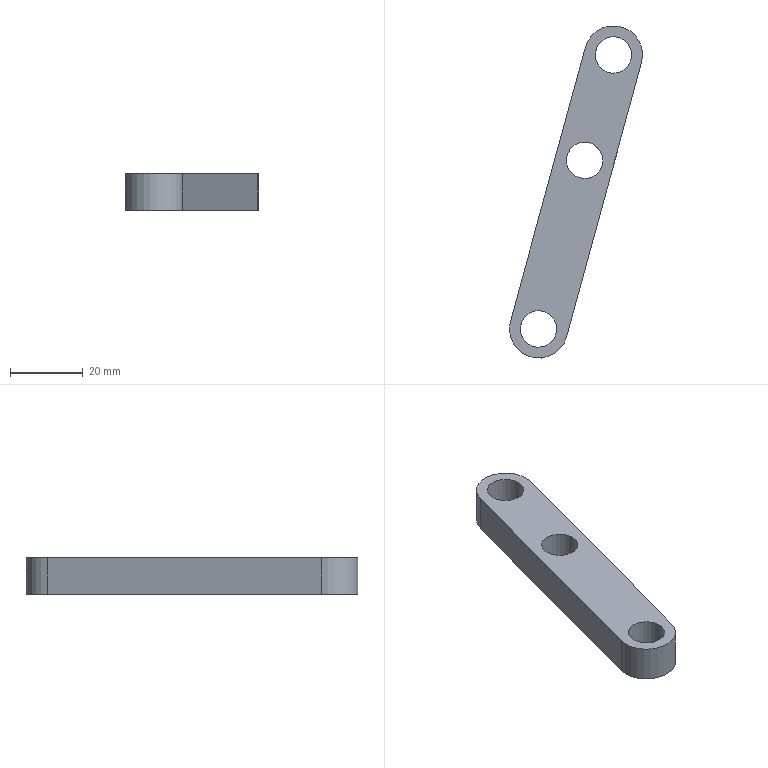Component | SolidWorks | ARocker-2 | 1 solid | 13 faces | box 36.56 x 91.24 x 10 mm | volume 12134 mm3 | cylinder 9 | plane 4 | commonest cylinder face diameters 10 x6 16 x3
build123d program:
from build123d import *

# Parameters (mm, degrees)
SKETCH1_R           = 5
BOSS_EXTRUDE1_DEPTH = 10


with BuildPart() as part:
    # Sketch1 → Boss-Extrude1 (new body)
    with BuildSketch(Plane.XY):
        with BuildLine():
            Line((-11.233, -5.015), (-60.126, 55.759))
            ThreePointArc((-60.126, 55.759), (-58.908, 67.007), (-47.66, 65.788))
            Line((-47.66, 65.788), (1.233, 5.015))
            ThreePointArc((1.233, 5.015), (0.01469, -6.233), (-11.233, -5.015))
        make_face()
        with Locations((-5, 0)):
            Circle(SKETCH1_R, mode=Mode.SUBTRACT)
        with Locations((-53.893, 60.774)):
            Circle(SKETCH1_R, mode=Mode.SUBTRACT)
        with Locations((-35.088, 37.399)):
            Circle(SKETCH1_R, mode=Mode.SUBTRACT)
    extrude(amount=BOSS_EXTRUDE1_DEPTH)


solid = part.part

# Placed as in the assembly
solid = solid.moved(Location((-69.375, -101.344, 137.182), (180, 0, 156.465)))
STEP:
#1=CARTESIAN_POINT('',(-2.168,-1.929,5.401));
#2=VERTEX_POINT('',#1);
#3=CARTESIAN_POINT('',(-1.937,-2.248,5.401));
#4=VERTEX_POINT('',#3);
#5=CARTESIAN_POINT('',(-2.053,-2.088,5.401));
#6=DIRECTION('',(-0.,0.,1.));
#7=DIRECTION('',(0.5864,-0.81,0.));
#8=AXIS2_PLACEMENT_3D('',#5,#6,#7);
#9=CIRCLE('',#8,0.1969);
#10=EDGE_CURVE('',#2,#4,#9,.T.);
#11=ORIENTED_EDGE('',*,*,#10,.T.);
#12=CARTESIAN_POINT('',(-1.937,-2.248,5.007));
#13=VERTEX_POINT('',#12);
#14=CARTESIAN_POINT('',(-1.937,-2.248,5.401));
#15=DIRECTION('',(0.,-0.,-1.));
#16=VECTOR('',#15,39.37);
#17=LINE('',#14,#16);
#18=EDGE_CURVE('',#4,#13,#17,.T.);
#19=ORIENTED_EDGE('',*,*,#18,.T.);
#20=CARTESIAN_POINT('',(-2.168,-1.929,5.007));
#21=VERTEX_POINT('',#20);
#22=CARTESIAN_POINT('',(-2.053,-2.088,5.007));
#23=DIRECTION('',(-0.,0.,1.));
#24=DIRECTION('',(0.5864,-0.81,0.));
#25=AXIS2_PLACEMENT_3D('',#22,#23,#24);
#26=CIRCLE('',#25,0.1969);
#27=EDGE_CURVE('',#21,#13,#26,.T.);
#28=ORIENTED_EDGE('',*,*,#27,.F.);
#29=CARTESIAN_POINT('',(-2.168,-1.929,5.401));
#30=DIRECTION('',(0.,-0.,-1.));
#31=VECTOR('',#30,39.37);
#32=LINE('',#29,#31);
#33=EDGE_CURVE('',#2,#21,#32,.T.);
#34=ORIENTED_EDGE('',*,*,#33,.F.);
#35=EDGE_LOOP('',(#11,#19,#28,#34));
#36=FACE_OUTER_BOUND('',#35,.T.);
#37=CARTESIAN_POINT('',(-2.053,-2.088,5.401));
#38=DIRECTION('',(0.,-0.,-1.));
#39=DIRECTION('',(-0.5864,0.81,0.));
#40=AXIS2_PLACEMENT_3D('',#37,#38,#39);
#41=CYLINDRICAL_SURFACE('',#40,0.1969);
#42=ADVANCED_FACE('',(#36),#41,.F.);
#43=CARTESIAN_POINT('',(-1.857,-0.7896,5.401));
#44=VERTEX_POINT('',#43);
#45=CARTESIAN_POINT('',(-1.626,-1.108,5.401));
#46=VERTEX_POINT('',#45);
#47=CARTESIAN_POINT('',(-1.741,-0.949,5.401));
#48=DIRECTION('',(-0.,0.,1.));
#49=DIRECTION('',(0.5864,-0.81,0.));
#50=AXIS2_PLACEMENT_3D('',#47,#48,#49);
#51=CIRCLE('',#50,0.1969);
#52=EDGE_CURVE('',#44,#46,#51,.T.);
#53=ORIENTED_EDGE('',*,*,#52,.T.);
#54=CARTESIAN_POINT('',(-1.626,-1.108,5.007));
#55=VERTEX_POINT('',#54);
#56=CARTESIAN_POINT('',(-1.626,-1.108,5.401));
#57=DIRECTION('',(0.,-0.,-1.));
#58=VECTOR('',#57,39.37);
#59=LINE('',#56,#58);
#60=EDGE_CURVE('',#46,#55,#59,.T.);
#61=ORIENTED_EDGE('',*,*,#60,.T.);
#62=CARTESIAN_POINT('',(-1.857,-0.7896,5.007));
#63=VERTEX_POINT('',#62);
#64=CARTESIAN_POINT('',(-1.741,-0.949,5.007));
#65=DIRECTION('',(-0.,0.,1.));
#66=DIRECTION('',(0.5864,-0.81,0.));
#67=AXIS2_PLACEMENT_3D('',#64,#65,#66);
#68=CIRCLE('',#67,0.1969);
#69=EDGE_CURVE('',#63,#55,#68,.T.);
#70=ORIENTED_EDGE('',*,*,#69,.F.);
#71=CARTESIAN_POINT('',(-1.857,-0.7896,5.401));
#72=DIRECTION('',(0.,-0.,-1.));
#73=VECTOR('',#72,39.37);
#74=LINE('',#71,#73);
#75=EDGE_CURVE('',#44,#63,#74,.T.);
#76=ORIENTED_EDGE('',*,*,#75,.F.);
#77=EDGE_LOOP('',(#53,#61,#70,#76));
#78=FACE_OUTER_BOUND('',#77,.T.);
#79=CARTESIAN_POINT('',(-1.741,-0.949,5.401));
#80=DIRECTION('',(0.,-0.,-1.));
#81=DIRECTION('',(-0.5864,0.81,0.));
#82=AXIS2_PLACEMENT_3D('',#79,#80,#81);
#83=CYLINDRICAL_SURFACE('',#82,0.1969);
#84=ADVANCED_FACE('',(#78),#83,.F.);
#85=CARTESIAN_POINT('',(-2.666,-3.752,5.401));
#86=VERTEX_POINT('',#85);
#87=CARTESIAN_POINT('',(-2.435,-4.071,5.401));
#88=VERTEX_POINT('',#87);
#89=CARTESIAN_POINT('',(-2.551,-3.911,5.401));
#90=DIRECTION('',(-0.,0.,1.));
#91=DIRECTION('',(0.5864,-0.81,0.));
#92=AXIS2_PLACEMENT_3D('',#89,#90,#91);
#93=CIRCLE('',#92,0.1969);
#94=EDGE_CURVE('',#86,#88,#93,.T.);
#95=ORIENTED_EDGE('',*,*,#94,.T.);
#96=CARTESIAN_POINT('',(-2.435,-4.071,5.007));
#97=VERTEX_POINT('',#96);
#98=CARTESIAN_POINT('',(-2.435,-4.071,5.401));
#99=DIRECTION('',(0.,-0.,-1.));
#100=VECTOR('',#99,39.37);
#101=LINE('',#98,#100);
#102=EDGE_CURVE('',#88,#97,#101,.T.);
#103=ORIENTED_EDGE('',*,*,#102,.T.);
#104=CARTESIAN_POINT('',(-2.666,-3.752,5.007));
#105=VERTEX_POINT('',#104);
#106=CARTESIAN_POINT('',(-2.551,-3.911,5.007));
#107=DIRECTION('',(-0.,0.,1.));
#108=DIRECTION('',(0.5864,-0.81,0.));
#109=AXIS2_PLACEMENT_3D('',#106,#107,#108);
#110=CIRCLE('',#109,0.1969);
#111=EDGE_CURVE('',#105,#97,#110,.T.);
#112=ORIENTED_EDGE('',*,*,#111,.F.);
#113=CARTESIAN_POINT('',(-2.666,-3.752,5.401));
#114=DIRECTION('',(0.,-0.,-1.));
#115=VECTOR('',#114,39.37);
#116=LINE('',#113,#115);
#117=EDGE_CURVE('',#86,#105,#116,.T.);
#118=ORIENTED_EDGE('',*,*,#117,.F.);
#119=EDGE_LOOP('',(#95,#103,#112,#118));
#120=FACE_OUTER_BOUND('',#119,.T.);
#121=CARTESIAN_POINT('',(-2.551,-3.911,5.401));
#122=DIRECTION('',(0.,-0.,-1.));
#123=DIRECTION('',(-0.5864,0.81,0.));
#124=AXIS2_PLACEMENT_3D('',#121,#122,#123);
#125=CYLINDRICAL_SURFACE('',#124,0.1969);
#126=ADVANCED_FACE('',(#120),#125,.F.);
#127=CARTESIAN_POINT('',(-1.926,-0.6939,5.401));
#128=VERTEX_POINT('',#127);
#129=CARTESIAN_POINT('',(-2.045,-0.866,5.401));
#130=VERTEX_POINT('',#129);
#131=CARTESIAN_POINT('',(-1.741,-0.949,5.401));
#132=DIRECTION('',(-0.,0.,1.));
#133=DIRECTION('',(0.5864,-0.81,0.));
#134=AXIS2_PLACEMENT_3D('',#131,#132,#133);
#135=CIRCLE('',#134,0.315);
#136=EDGE_CURVE('',#128,#130,#135,.T.);
#137=ORIENTED_EDGE('',*,*,#136,.F.);
#138=CARTESIAN_POINT('',(-1.926,-0.6939,5.007));
#139=VERTEX_POINT('',#138);
#140=CARTESIAN_POINT('',(-1.926,-0.6939,5.401));
#141=DIRECTION('',(0.,-0.,-1.));
#142=VECTOR('',#141,39.37);
#143=LINE('',#140,#142);
#144=EDGE_CURVE('',#128,#139,#143,.T.);
#145=ORIENTED_EDGE('',*,*,#144,.T.);
#146=CARTESIAN_POINT('',(-2.045,-0.866,5.007));
#147=VERTEX_POINT('',#146);
#148=CARTESIAN_POINT('',(-1.741,-0.949,5.007));
#149=DIRECTION('',(-0.,0.,1.));
#150=DIRECTION('',(0.5864,-0.81,0.));
#151=AXIS2_PLACEMENT_3D('',#148,#149,#150);
#152=CIRCLE('',#151,0.315);
#153=EDGE_CURVE('',#139,#147,#152,.T.);
#154=ORIENTED_EDGE('',*,*,#153,.T.);
#155=CARTESIAN_POINT('',(-2.045,-0.866,5.401));
#156=DIRECTION('',(0.,-0.,-1.));
#157=VECTOR('',#156,39.37);
#158=LINE('',#155,#157);
#159=EDGE_CURVE('',#130,#147,#158,.T.);
#160=ORIENTED_EDGE('',*,*,#159,.F.);
#161=EDGE_LOOP('',(#137,#145,#154,#160));
#162=FACE_OUTER_BOUND('',#161,.T.);
#163=CARTESIAN_POINT('',(-1.741,-0.949,5.401));
#164=DIRECTION('',(0.,-0.,-1.));
#165=DIRECTION('',(-0.5864,0.81,0.));
#166=AXIS2_PLACEMENT_3D('',#163,#164,#165);
#167=CYLINDRICAL_SURFACE('',#166,0.315);
#168=ADVANCED_FACE('',(#162),#167,.T.);
#169=ORIENTED_EDGE('',*,*,#52,.F.);
#170=CARTESIAN_POINT('',(-1.741,-0.949,5.401));
#171=DIRECTION('',(-0.,0.,1.));
#172=DIRECTION('',(0.5864,-0.81,0.));
#173=AXIS2_PLACEMENT_3D('',#170,#171,#172);
#174=CIRCLE('',#173,0.1969);
#175=EDGE_CURVE('',#46,#44,#174,.T.);
#176=ORIENTED_EDGE('',*,*,#175,.F.);
#177=EDGE_LOOP('',(#169,#176));
#178=FACE_BOUND('',#177,.T.);
#179=CARTESIAN_POINT('',(-2.855,-3.828,5.401));
#180=VERTEX_POINT('',#179);
#181=CARTESIAN_POINT('',(-2.247,-3.994,5.401));
#182=VERTEX_POINT('',#181);
#183=CARTESIAN_POINT('',(-2.551,-3.911,5.401));
#184=DIRECTION('',(-0.,0.,1.));
#185=DIRECTION('',(0.5864,-0.81,0.));
#186=AXIS2_PLACEMENT_3D('',#183,#184,#185);
#187=CIRCLE('',#186,0.315);
#188=EDGE_CURVE('',#180,#182,#187,.T.);
#189=ORIENTED_EDGE('',*,*,#188,.T.);
#190=CARTESIAN_POINT('',(-1.438,-1.032,5.401));
#191=VERTEX_POINT('',#190);
#192=CARTESIAN_POINT('',(-2.247,-3.994,5.401));
#193=DIRECTION('',(0.2636,0.9646,-0.));
#194=VECTOR('',#193,39.37);
#195=LINE('',#192,#194);
#196=EDGE_CURVE('',#182,#191,#195,.T.);
#197=ORIENTED_EDGE('',*,*,#196,.T.);
#198=CARTESIAN_POINT('',(-1.741,-0.949,5.401));
#199=DIRECTION('',(-0.,0.,1.));
#200=DIRECTION('',(0.5864,-0.81,0.));
#201=AXIS2_PLACEMENT_3D('',#198,#199,#200);
#202=CIRCLE('',#201,0.315);
#203=EDGE_CURVE('',#191,#128,#202,.T.);
#204=ORIENTED_EDGE('',*,*,#203,.T.);
#205=ORIENTED_EDGE('',*,*,#136,.T.);
#206=CARTESIAN_POINT('',(-2.855,-3.828,5.401));
#207=DIRECTION('',(-0.2636,-0.9646,0.));
#208=VECTOR('',#207,39.37);
#209=LINE('',#206,#208);
#210=EDGE_CURVE('',#130,#180,#209,.T.);
#211=ORIENTED_EDGE('',*,*,#210,.T.);
#212=EDGE_LOOP('',(#189,#197,#204,#205,#211));
#213=FACE_OUTER_BOUND('',#212,.T.);
#214=ORIENTED_EDGE('',*,*,#94,.F.);
#215=CARTESIAN_POINT('',(-2.551,-3.911,5.401));
#216=DIRECTION('',(-0.,0.,1.));
#217=DIRECTION('',(0.5864,-0.81,0.));
#218=AXIS2_PLACEMENT_3D('',#215,#216,#217);
#219=CIRCLE('',#218,0.1969);
#220=EDGE_CURVE('',#88,#86,#219,.T.);
#221=ORIENTED_EDGE('',*,*,#220,.F.);
#222=EDGE_LOOP('',(#214,#221));
#223=FACE_BOUND('',#222,.T.);
#224=ORIENTED_EDGE('',*,*,#10,.F.);
#225=CARTESIAN_POINT('',(-2.053,-2.088,5.401));
#226=DIRECTION('',(-0.,0.,1.));
#227=DIRECTION('',(0.5864,-0.81,0.));
#228=AXIS2_PLACEMENT_3D('',#225,#226,#227);
#229=CIRCLE('',#228,0.1969);
#230=EDGE_CURVE('',#4,#2,#229,.T.);
#231=ORIENTED_EDGE('',*,*,#230,.F.);
#232=EDGE_LOOP('',(#224,#231));
#233=FACE_BOUND('',#232,.T.);
#234=CARTESIAN_POINT('',(-2.551,-3.911,5.401));
#235=DIRECTION('',(-0.,0.,1.));
#236=DIRECTION('',(0.5864,-0.81,0.));
#237=AXIS2_PLACEMENT_3D('',#234,#235,#236);
#238=PLANE('',#237);
#239=ADVANCED_FACE('',(#178,#213,#223,#233),#238,.T.);
#240=CARTESIAN_POINT('',(-2.855,-3.828,5.007));
#241=VERTEX_POINT('',#240);
#242=CARTESIAN_POINT('',(-2.247,-3.994,5.007));
#243=VERTEX_POINT('',#242);
#244=CARTESIAN_POINT('',(-2.551,-3.911,5.007));
#245=DIRECTION('',(-0.,0.,1.));
#246=DIRECTION('',(0.5864,-0.81,0.));
#247=AXIS2_PLACEMENT_3D('',#244,#245,#246);
#248=CIRCLE('',#247,0.315);
#249=EDGE_CURVE('',#241,#243,#248,.T.);
#250=ORIENTED_EDGE('',*,*,#249,.F.);
#251=CARTESIAN_POINT('',(-2.855,-3.828,5.007));
#252=DIRECTION('',(-0.2636,-0.9646,0.));
#253=VECTOR('',#252,39.37);
#254=LINE('',#251,#253);
#255=EDGE_CURVE('',#147,#241,#254,.T.);
#256=ORIENTED_EDGE('',*,*,#255,.F.);
#257=ORIENTED_EDGE('',*,*,#153,.F.);
#258=CARTESIAN_POINT('',(-1.438,-1.032,5.007));
#259=VERTEX_POINT('',#258);
#260=CARTESIAN_POINT('',(-1.741,-0.949,5.007));
#261=DIRECTION('',(-0.,0.,1.));
#262=DIRECTION('',(0.5864,-0.81,0.));
#263=AXIS2_PLACEMENT_3D('',#260,#261,#262);
#264=CIRCLE('',#263,0.315);
#265=EDGE_CURVE('',#259,#139,#264,.T.);
#266=ORIENTED_EDGE('',*,*,#265,.F.);
#267=CARTESIAN_POINT('',(-2.247,-3.994,5.007));
#268=DIRECTION('',(0.2636,0.9646,-0.));
#269=VECTOR('',#268,39.37);
#270=LINE('',#267,#269);
#271=EDGE_CURVE('',#243,#259,#270,.T.);
#272=ORIENTED_EDGE('',*,*,#271,.F.);
#273=EDGE_LOOP('',(#250,#256,#257,#266,#272));
#274=FACE_OUTER_BOUND('',#273,.T.);
#275=ORIENTED_EDGE('',*,*,#111,.T.);
#276=CARTESIAN_POINT('',(-2.551,-3.911,5.007));
#277=DIRECTION('',(-0.,0.,1.));
#278=DIRECTION('',(0.5864,-0.81,0.));
#279=AXIS2_PLACEMENT_3D('',#276,#277,#278);
#280=CIRCLE('',#279,0.1969);
#281=EDGE_CURVE('',#97,#105,#280,.T.);
#282=ORIENTED_EDGE('',*,*,#281,.T.);
#283=EDGE_LOOP('',(#275,#282));
#284=FACE_BOUND('',#283,.T.);
#285=ORIENTED_EDGE('',*,*,#69,.T.);
#286=CARTESIAN_POINT('',(-1.741,-0.949,5.007));
#287=DIRECTION('',(-0.,0.,1.));
#288=DIRECTION('',(0.5864,-0.81,0.));
#289=AXIS2_PLACEMENT_3D('',#286,#287,#288);
#290=CIRCLE('',#289,0.1969);
#291=EDGE_CURVE('',#55,#63,#290,.T.);
#292=ORIENTED_EDGE('',*,*,#291,.T.);
#293=EDGE_LOOP('',(#285,#292));
#294=FACE_BOUND('',#293,.T.);
#295=ORIENTED_EDGE('',*,*,#27,.T.);
#296=CARTESIAN_POINT('',(-2.053,-2.088,5.007));
#297=DIRECTION('',(-0.,0.,1.));
#298=DIRECTION('',(0.5864,-0.81,0.));
#299=AXIS2_PLACEMENT_3D('',#296,#297,#298);
#300=CIRCLE('',#299,0.1969);
#301=EDGE_CURVE('',#13,#21,#300,.T.);
#302=ORIENTED_EDGE('',*,*,#301,.T.);
#303=EDGE_LOOP('',(#295,#302));
#304=FACE_BOUND('',#303,.T.);
#305=CARTESIAN_POINT('',(-2.551,-3.911,5.007));
#306=DIRECTION('',(-0.,0.,1.));
#307=DIRECTION('',(0.5864,-0.81,0.));
#308=AXIS2_PLACEMENT_3D('',#305,#306,#307);
#309=PLANE('',#308);
#310=ADVANCED_FACE('',(#274,#284,#294,#304),#309,.F.);
#311=ORIENTED_EDGE('',*,*,#249,.T.);
#312=CARTESIAN_POINT('',(-2.247,-3.994,5.401));
#313=DIRECTION('',(0.,-0.,-1.));
#314=VECTOR('',#313,39.37);
#315=LINE('',#312,#314);
#316=EDGE_CURVE('',#182,#243,#315,.T.);
#317=ORIENTED_EDGE('',*,*,#316,.F.);
#318=ORIENTED_EDGE('',*,*,#188,.F.);
#319=CARTESIAN_POINT('',(-2.855,-3.828,5.401));
#320=DIRECTION('',(0.,-0.,-1.));
#321=VECTOR('',#320,39.37);
#322=LINE('',#319,#321);
#323=EDGE_CURVE('',#180,#241,#322,.T.);
#324=ORIENTED_EDGE('',*,*,#323,.T.);
#325=EDGE_LOOP('',(#311,#317,#318,#324));
#326=FACE_OUTER_BOUND('',#325,.T.);
#327=CARTESIAN_POINT('',(-2.551,-3.911,5.401));
#328=DIRECTION('',(0.,-0.,-1.));
#329=DIRECTION('',(-0.5864,0.81,0.));
#330=AXIS2_PLACEMENT_3D('',#327,#328,#329);
#331=CYLINDRICAL_SURFACE('',#330,0.315);
#332=ADVANCED_FACE('',(#326),#331,.T.);
#333=ORIENTED_EDGE('',*,*,#271,.T.);
#334=CARTESIAN_POINT('',(-1.438,-1.032,5.401));
#335=DIRECTION('',(0.,-0.,-1.));
#336=VECTOR('',#335,39.37);
#337=LINE('',#334,#336);
#338=EDGE_CURVE('',#191,#259,#337,.T.);
#339=ORIENTED_EDGE('',*,*,#338,.F.);
#340=ORIENTED_EDGE('',*,*,#196,.F.);
#341=ORIENTED_EDGE('',*,*,#316,.T.);
#342=EDGE_LOOP('',(#333,#339,#340,#341));
#343=FACE_OUTER_BOUND('',#342,.T.);
#344=CARTESIAN_POINT('',(-2.247,-3.994,5.401));
#345=DIRECTION('',(-0.9646,0.2636,-0.));
#346=DIRECTION('',(-0.2636,-0.9646,0.));
#347=AXIS2_PLACEMENT_3D('',#344,#345,#346);
#348=PLANE('',#347);
#349=ADVANCED_FACE('',(#343),#348,.F.);
#350=ORIENTED_EDGE('',*,*,#144,.F.);
#351=ORIENTED_EDGE('',*,*,#203,.F.);
#352=ORIENTED_EDGE('',*,*,#338,.T.);
#353=ORIENTED_EDGE('',*,*,#265,.T.);
#354=EDGE_LOOP('',(#350,#351,#352,#353));
#355=FACE_OUTER_BOUND('',#354,.T.);
#356=CARTESIAN_POINT('',(-1.741,-0.949,5.401));
#357=DIRECTION('',(0.,-0.,-1.));
#358=DIRECTION('',(-0.5864,0.81,0.));
#359=AXIS2_PLACEMENT_3D('',#356,#357,#358);
#360=CYLINDRICAL_SURFACE('',#359,0.315);
#361=ADVANCED_FACE('',(#355),#360,.T.);
#362=ORIENTED_EDGE('',*,*,#255,.T.);
#363=ORIENTED_EDGE('',*,*,#323,.F.);
#364=ORIENTED_EDGE('',*,*,#210,.F.);
#365=ORIENTED_EDGE('',*,*,#159,.T.);
#366=EDGE_LOOP('',(#362,#363,#364,#365));
#367=FACE_OUTER_BOUND('',#366,.T.);
#368=CARTESIAN_POINT('',(-2.855,-3.828,5.401));
#369=DIRECTION('',(0.9646,-0.2636,0.));
#370=DIRECTION('',(0.2636,0.9646,-0.));
#371=AXIS2_PLACEMENT_3D('',#368,#369,#370);
#372=PLANE('',#371);
#373=ADVANCED_FACE('',(#367),#372,.F.);
#374=ORIENTED_EDGE('',*,*,#102,.F.);
#375=ORIENTED_EDGE('',*,*,#220,.T.);
#376=ORIENTED_EDGE('',*,*,#117,.T.);
#377=ORIENTED_EDGE('',*,*,#281,.F.);
#378=EDGE_LOOP('',(#374,#375,#376,#377));
#379=FACE_OUTER_BOUND('',#378,.T.);
#380=CARTESIAN_POINT('',(-2.551,-3.911,5.401));
#381=DIRECTION('',(0.,-0.,-1.));
#382=DIRECTION('',(-0.5864,0.81,0.));
#383=AXIS2_PLACEMENT_3D('',#380,#381,#382);
#384=CYLINDRICAL_SURFACE('',#383,0.1969);
#385=ADVANCED_FACE('',(#379),#384,.F.);
#386=ORIENTED_EDGE('',*,*,#60,.F.);
#387=ORIENTED_EDGE('',*,*,#175,.T.);
#388=ORIENTED_EDGE('',*,*,#75,.T.);
#389=ORIENTED_EDGE('',*,*,#291,.F.);
#390=EDGE_LOOP('',(#386,#387,#388,#389));
#391=FACE_OUTER_BOUND('',#390,.T.);
#392=CARTESIAN_POINT('',(-1.741,-0.949,5.401));
#393=DIRECTION('',(0.,-0.,-1.));
#394=DIRECTION('',(-0.5864,0.81,0.));
#395=AXIS2_PLACEMENT_3D('',#392,#393,#394);
#396=CYLINDRICAL_SURFACE('',#395,0.1969);
#397=ADVANCED_FACE('',(#391),#396,.F.);
#398=ORIENTED_EDGE('',*,*,#18,.F.);
#399=ORIENTED_EDGE('',*,*,#230,.T.);
#400=ORIENTED_EDGE('',*,*,#33,.T.);
#401=ORIENTED_EDGE('',*,*,#301,.F.);
#402=EDGE_LOOP('',(#398,#399,#400,#401));
#403=FACE_OUTER_BOUND('',#402,.T.);
#404=CARTESIAN_POINT('',(-2.053,-2.088,5.401));
#405=DIRECTION('',(0.,-0.,-1.));
#406=DIRECTION('',(-0.5864,0.81,0.));
#407=AXIS2_PLACEMENT_3D('',#404,#405,#406);
#408=CYLINDRICAL_SURFACE('',#407,0.1969);
#409=ADVANCED_FACE('',(#403),#408,.F.);
#410=CLOSED_SHELL('',(#42,#84,#126,#168,#239,#310,#332,#349,#361,#373,#385,#397,#409));
#411=MANIFOLD_SOLID_BREP('',#410);
#412=CARTESIAN_POINT('',(0.,0.,0.));
#413=DIRECTION('',(0.,0.,1.));
#414=DIRECTION('',(1.,0.,0.));
#415=AXIS2_PLACEMENT_3D('',#412,#413,#414);
#416=(LENGTH_UNIT()NAMED_UNIT(*)SI_UNIT($,.METRE.));
#417=LENGTH_MEASURE_WITH_UNIT(LENGTH_MEASURE(0.0254),#416);
#418=DIMENSIONAL_EXPONENTS(1.,0.,0.,0.,0.,0.,0.);
#419=(CONVERSION_BASED_UNIT('',#417)LENGTH_UNIT()NAMED_UNIT(#418));
#420=UNCERTAINTY_MEASURE_WITH_UNIT(LENGTH_MEASURE(0.00001),#419,'','');
#421=(NAMED_UNIT(*)PLANE_ANGLE_UNIT()SI_UNIT($,.RADIAN.));
#422=(NAMED_UNIT(*)SI_UNIT($,.STERADIAN.)SOLID_ANGLE_UNIT());
#423=(GEOMETRIC_REPRESENTATION_CONTEXT(3)GLOBAL_UNCERTAINTY_ASSIGNED_CONTEXT((#420))GLOBAL_UNIT_ASSIGNED_CONTEXT((#419,#421,#422))REPRESENTATION_CONTEXT('',''));
#424=ADVANCED_BREP_SHAPE_REPRESENTATION('',(#411,#415),#423);
#425=COLOUR_RGB('',0.7922,0.8196,0.9333);
#426=FILL_AREA_STYLE_COLOUR('',#425);
#427=FILL_AREA_STYLE('',(#426));
#428=SURFACE_STYLE_FILL_AREA(#427);
#429=SURFACE_SIDE_STYLE('',(#428));
#430=SURFACE_STYLE_USAGE(.BOTH.,#429);
#431=PRESENTATION_STYLE_ASSIGNMENT((#430));
#432=STYLED_ITEM('',(#431),#411);
#433=PRESENTATION_LAYER_ASSIGNMENT('','',(#432));
#434=(LENGTH_UNIT()NAMED_UNIT(*)SI_UNIT($,.METRE.));
#435=LENGTH_MEASURE_WITH_UNIT(LENGTH_MEASURE(0.0254),#434);
#436=DIMENSIONAL_EXPONENTS(1.,0.,0.,0.,0.,0.,0.);
#437=(CONVERSION_BASED_UNIT('',#435)LENGTH_UNIT()NAMED_UNIT(#436));
#438=UNCERTAINTY_MEASURE_WITH_UNIT(LENGTH_MEASURE(0.00001),#437,'','');
#439=(NAMED_UNIT(*)PLANE_ANGLE_UNIT()SI_UNIT($,.RADIAN.));
#440=(NAMED_UNIT(*)SI_UNIT($,.STERADIAN.)SOLID_ANGLE_UNIT());
#441=(GEOMETRIC_REPRESENTATION_CONTEXT(3)GLOBAL_UNCERTAINTY_ASSIGNED_CONTEXT((#438))GLOBAL_UNIT_ASSIGNED_CONTEXT((#437,#439,#440))REPRESENTATION_CONTEXT('',''));
#442=MECHANICAL_DESIGN_GEOMETRIC_PRESENTATION_REPRESENTATION('',(#432),#441);